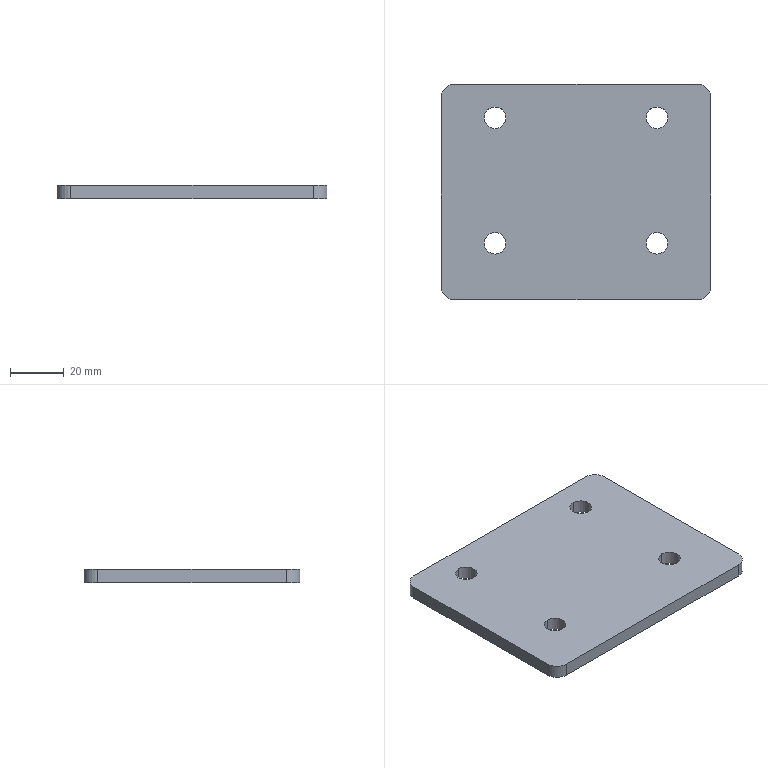Component | SolidWorks | VerticalMovingRectangularTubeWeldment-1_RectangularTubeWeldPlate1-2 | 1 solid | 18 faces | box 100 x 80 x 5 mm | volume 38887 mm3 | cylinder 12 | plane 6 | commonest cylinder face diameters 8 x8 10 x4 | material Plain Carbon Steel
STEP:
#1=CARTESIAN_POINT('',(11.024,-0.9055,-0.7874));
#2=VERTEX_POINT('',#1);
#3=CARTESIAN_POINT('',(11.024,-0.5906,-0.7874));
#4=VERTEX_POINT('',#3);
#5=CARTESIAN_POINT('',(11.024,-0.748,-0.7874));
#6=DIRECTION('',(0.,0.,-1.));
#7=DIRECTION('',(0.,1.,0.));
#8=AXIS2_PLACEMENT_3D('',#5,#6,#7);
#9=CIRCLE('',#8,0.1575);
#10=EDGE_CURVE('',#2,#4,#9,.T.);
#11=ORIENTED_EDGE('',*,*,#10,.F.);
#12=CARTESIAN_POINT('',(11.024,-0.9055,-0.9843));
#13=VERTEX_POINT('',#12);
#14=CARTESIAN_POINT('',(11.024,-0.9055,-0.9843));
#15=DIRECTION('',(0.,-0.,-1.));
#16=VECTOR('',#15,39.37);
#17=LINE('',#14,#16);
#18=EDGE_CURVE('',#2,#13,#17,.T.);
#19=ORIENTED_EDGE('',*,*,#18,.T.);
#20=CARTESIAN_POINT('',(11.024,-0.5906,-0.9843));
#21=VERTEX_POINT('',#20);
#22=CARTESIAN_POINT('',(11.024,-0.748,-0.9843));
#23=DIRECTION('',(0.,-0.,-1.));
#24=DIRECTION('',(0.,1.,0.));
#25=AXIS2_PLACEMENT_3D('',#22,#23,#24);
#26=CIRCLE('',#25,0.1575);
#27=EDGE_CURVE('',#13,#21,#26,.T.);
#28=ORIENTED_EDGE('',*,*,#27,.T.);
#29=CARTESIAN_POINT('',(11.024,-0.5906,-0.9843));
#30=DIRECTION('',(0.,-0.,-1.));
#31=VECTOR('',#30,39.37);
#32=LINE('',#29,#31);
#33=EDGE_CURVE('',#4,#21,#32,.T.);
#34=ORIENTED_EDGE('',*,*,#33,.F.);
#35=EDGE_LOOP('',(#11,#19,#28,#34));
#36=FACE_OUTER_BOUND('',#35,.T.);
#37=CARTESIAN_POINT('',(11.024,-0.748,-0.9843));
#38=DIRECTION('',(0.,-0.,-1.));
#39=DIRECTION('',(0.,1.,0.));
#40=AXIS2_PLACEMENT_3D('',#37,#38,#39);
#41=CYLINDRICAL_SURFACE('',#40,0.1575);
#42=ADVANCED_FACE('',(#36),#41,.F.);
#43=CARTESIAN_POINT('',(8.661,-0.9055,-0.7874));
#44=VERTEX_POINT('',#43);
#45=CARTESIAN_POINT('',(8.661,-0.5906,-0.7874));
#46=VERTEX_POINT('',#45);
#47=CARTESIAN_POINT('',(8.661,-0.748,-0.7874));
#48=DIRECTION('',(0.,0.,-1.));
#49=DIRECTION('',(0.,1.,0.));
#50=AXIS2_PLACEMENT_3D('',#47,#48,#49);
#51=CIRCLE('',#50,0.1575);
#52=EDGE_CURVE('',#44,#46,#51,.T.);
#53=ORIENTED_EDGE('',*,*,#52,.F.);
#54=CARTESIAN_POINT('',(8.661,-0.9055,-0.9843));
#55=VERTEX_POINT('',#54);
#56=CARTESIAN_POINT('',(8.661,-0.9055,-0.9843));
#57=DIRECTION('',(0.,-0.,-1.));
#58=VECTOR('',#57,39.37);
#59=LINE('',#56,#58);
#60=EDGE_CURVE('',#44,#55,#59,.T.);
#61=ORIENTED_EDGE('',*,*,#60,.T.);
#62=CARTESIAN_POINT('',(8.661,-0.5906,-0.9843));
#63=VERTEX_POINT('',#62);
#64=CARTESIAN_POINT('',(8.661,-0.748,-0.9843));
#65=DIRECTION('',(0.,-0.,-1.));
#66=DIRECTION('',(0.,1.,0.));
#67=AXIS2_PLACEMENT_3D('',#64,#65,#66);
#68=CIRCLE('',#67,0.1575);
#69=EDGE_CURVE('',#55,#63,#68,.T.);
#70=ORIENTED_EDGE('',*,*,#69,.T.);
#71=CARTESIAN_POINT('',(8.661,-0.5906,-0.9843));
#72=DIRECTION('',(0.,-0.,-1.));
#73=VECTOR('',#72,39.37);
#74=LINE('',#71,#73);
#75=EDGE_CURVE('',#46,#63,#74,.T.);
#76=ORIENTED_EDGE('',*,*,#75,.F.);
#77=EDGE_LOOP('',(#53,#61,#70,#76));
#78=FACE_OUTER_BOUND('',#77,.T.);
#79=CARTESIAN_POINT('',(8.661,-0.748,-0.9843));
#80=DIRECTION('',(0.,-0.,-1.));
#81=DIRECTION('',(0.,1.,0.));
#82=AXIS2_PLACEMENT_3D('',#79,#80,#81);
#83=CYLINDRICAL_SURFACE('',#82,0.1575);
#84=ADVANCED_FACE('',(#78),#83,.F.);
#85=CARTESIAN_POINT('',(11.024,0.9252,-0.7874));
#86=VERTEX_POINT('',#85);
#87=CARTESIAN_POINT('',(11.024,1.24,-0.7874));
#88=VERTEX_POINT('',#87);
#89=CARTESIAN_POINT('',(11.024,1.083,-0.7874));
#90=DIRECTION('',(0.,0.,-1.));
#91=DIRECTION('',(0.,1.,0.));
#92=AXIS2_PLACEMENT_3D('',#89,#90,#91);
#93=CIRCLE('',#92,0.1575);
#94=EDGE_CURVE('',#86,#88,#93,.T.);
#95=ORIENTED_EDGE('',*,*,#94,.F.);
#96=CARTESIAN_POINT('',(11.024,0.9252,-0.9843));
#97=VERTEX_POINT('',#96);
#98=CARTESIAN_POINT('',(11.024,0.9252,-0.9843));
#99=DIRECTION('',(0.,-0.,-1.));
#100=VECTOR('',#99,39.37);
#101=LINE('',#98,#100);
#102=EDGE_CURVE('',#86,#97,#101,.T.);
#103=ORIENTED_EDGE('',*,*,#102,.T.);
#104=CARTESIAN_POINT('',(11.024,1.24,-0.9843));
#105=VERTEX_POINT('',#104);
#106=CARTESIAN_POINT('',(11.024,1.083,-0.9843));
#107=DIRECTION('',(0.,-0.,-1.));
#108=DIRECTION('',(0.,1.,0.));
#109=AXIS2_PLACEMENT_3D('',#106,#107,#108);
#110=CIRCLE('',#109,0.1575);
#111=EDGE_CURVE('',#97,#105,#110,.T.);
#112=ORIENTED_EDGE('',*,*,#111,.T.);
#113=CARTESIAN_POINT('',(11.024,1.24,-0.9843));
#114=DIRECTION('',(0.,-0.,-1.));
#115=VECTOR('',#114,39.37);
#116=LINE('',#113,#115);
#117=EDGE_CURVE('',#88,#105,#116,.T.);
#118=ORIENTED_EDGE('',*,*,#117,.F.);
#119=EDGE_LOOP('',(#95,#103,#112,#118));
#120=FACE_OUTER_BOUND('',#119,.T.);
#121=CARTESIAN_POINT('',(11.024,1.083,-0.9843));
#122=DIRECTION('',(0.,-0.,-1.));
#123=DIRECTION('',(0.,1.,0.));
#124=AXIS2_PLACEMENT_3D('',#121,#122,#123);
#125=CYLINDRICAL_SURFACE('',#124,0.1575);
#126=ADVANCED_FACE('',(#120),#125,.F.);
#127=CARTESIAN_POINT('',(8.661,0.9252,-0.7874));
#128=VERTEX_POINT('',#127);
#129=CARTESIAN_POINT('',(8.661,1.24,-0.7874));
#130=VERTEX_POINT('',#129);
#131=CARTESIAN_POINT('',(8.661,1.083,-0.7874));
#132=DIRECTION('',(0.,0.,-1.));
#133=DIRECTION('',(0.,1.,0.));
#134=AXIS2_PLACEMENT_3D('',#131,#132,#133);
#135=CIRCLE('',#134,0.1575);
#136=EDGE_CURVE('',#128,#130,#135,.T.);
#137=ORIENTED_EDGE('',*,*,#136,.F.);
#138=CARTESIAN_POINT('',(8.661,0.9252,-0.9843));
#139=VERTEX_POINT('',#138);
#140=CARTESIAN_POINT('',(8.661,0.9252,-0.9843));
#141=DIRECTION('',(0.,-0.,-1.));
#142=VECTOR('',#141,39.37);
#143=LINE('',#140,#142);
#144=EDGE_CURVE('',#128,#139,#143,.T.);
#145=ORIENTED_EDGE('',*,*,#144,.T.);
#146=CARTESIAN_POINT('',(8.661,1.24,-0.9843));
#147=VERTEX_POINT('',#146);
#148=CARTESIAN_POINT('',(8.661,1.083,-0.9843));
#149=DIRECTION('',(0.,-0.,-1.));
#150=DIRECTION('',(0.,1.,0.));
#151=AXIS2_PLACEMENT_3D('',#148,#149,#150);
#152=CIRCLE('',#151,0.1575);
#153=EDGE_CURVE('',#139,#147,#152,.T.);
#154=ORIENTED_EDGE('',*,*,#153,.T.);
#155=CARTESIAN_POINT('',(8.661,1.24,-0.9843));
#156=DIRECTION('',(0.,-0.,-1.));
#157=VECTOR('',#156,39.37);
#158=LINE('',#155,#157);
#159=EDGE_CURVE('',#130,#147,#158,.T.);
#160=ORIENTED_EDGE('',*,*,#159,.F.);
#161=EDGE_LOOP('',(#137,#145,#154,#160));
#162=FACE_OUTER_BOUND('',#161,.T.);
#163=CARTESIAN_POINT('',(8.661,1.083,-0.9843));
#164=DIRECTION('',(0.,-0.,-1.));
#165=DIRECTION('',(0.,1.,0.));
#166=AXIS2_PLACEMENT_3D('',#163,#164,#165);
#167=CYLINDRICAL_SURFACE('',#166,0.1575);
#168=ADVANCED_FACE('',(#162),#167,.F.);
#169=CARTESIAN_POINT('',(11.811,-1.378,-0.7874));
#170=VERTEX_POINT('',#169);
#171=CARTESIAN_POINT('',(11.811,-1.378,-0.9843));
#172=VERTEX_POINT('',#171);
#173=CARTESIAN_POINT('',(11.811,-1.378,-0.7874));
#174=DIRECTION('',(0.,0.,-1.));
#175=VECTOR('',#174,39.37);
#176=LINE('',#173,#175);
#177=EDGE_CURVE('',#170,#172,#176,.T.);
#178=ORIENTED_EDGE('',*,*,#177,.T.);
#179=CARTESIAN_POINT('',(11.811,1.378,-0.9843));
#180=VERTEX_POINT('',#179);
#181=CARTESIAN_POINT('',(11.811,-1.575,-0.9843));
#182=DIRECTION('',(0.,1.,-0.));
#183=VECTOR('',#182,39.37);
#184=LINE('',#181,#183);
#185=EDGE_CURVE('',#172,#180,#184,.T.);
#186=ORIENTED_EDGE('',*,*,#185,.T.);
#187=CARTESIAN_POINT('',(11.811,1.378,-0.7874));
#188=VERTEX_POINT('',#187);
#189=CARTESIAN_POINT('',(11.811,1.378,-0.7874));
#190=DIRECTION('',(0.,0.,1.));
#191=VECTOR('',#190,39.37);
#192=LINE('',#189,#191);
#193=EDGE_CURVE('',#180,#188,#192,.T.);
#194=ORIENTED_EDGE('',*,*,#193,.T.);
#195=CARTESIAN_POINT('',(11.811,-1.575,-0.7874));
#196=DIRECTION('',(0.,1.,0.));
#197=VECTOR('',#196,39.37);
#198=LINE('',#195,#197);
#199=EDGE_CURVE('',#170,#188,#198,.T.);
#200=ORIENTED_EDGE('',*,*,#199,.F.);
#201=EDGE_LOOP('',(#178,#186,#194,#200));
#202=FACE_OUTER_BOUND('',#201,.T.);
#203=CARTESIAN_POINT('',(11.811,-1.575,-0.7874));
#204=DIRECTION('',(-1.,0.,0.));
#205=DIRECTION('',(0.,-1.,0.));
#206=AXIS2_PLACEMENT_3D('',#203,#204,#205);
#207=PLANE('',#206);
#208=ADVANCED_FACE('',(#202),#207,.F.);
#209=CARTESIAN_POINT('',(11.614,1.575,-0.7874));
#210=VERTEX_POINT('',#209);
#211=CARTESIAN_POINT('',(11.614,1.575,-0.9843));
#212=VERTEX_POINT('',#211);
#213=CARTESIAN_POINT('',(11.614,1.575,-0.7874));
#214=DIRECTION('',(0.,0.,-1.));
#215=VECTOR('',#214,39.37);
#216=LINE('',#213,#215);
#217=EDGE_CURVE('',#210,#212,#216,.T.);
#218=ORIENTED_EDGE('',*,*,#217,.T.);
#219=CARTESIAN_POINT('',(8.071,1.575,-0.9843));
#220=VERTEX_POINT('',#219);
#221=CARTESIAN_POINT('',(7.874,1.575,-0.9843));
#222=DIRECTION('',(-1.,0.,0.));
#223=VECTOR('',#222,39.37);
#224=LINE('',#221,#223);
#225=EDGE_CURVE('',#212,#220,#224,.T.);
#226=ORIENTED_EDGE('',*,*,#225,.T.);
#227=CARTESIAN_POINT('',(8.071,1.575,-0.7874));
#228=VERTEX_POINT('',#227);
#229=CARTESIAN_POINT('',(8.071,1.575,-0.7874));
#230=DIRECTION('',(0.,0.,1.));
#231=VECTOR('',#230,39.37);
#232=LINE('',#229,#231);
#233=EDGE_CURVE('',#220,#228,#232,.T.);
#234=ORIENTED_EDGE('',*,*,#233,.T.);
#235=CARTESIAN_POINT('',(7.874,1.575,-0.7874));
#236=DIRECTION('',(-1.,0.,0.));
#237=VECTOR('',#236,39.37);
#238=LINE('',#235,#237);
#239=EDGE_CURVE('',#210,#228,#238,.T.);
#240=ORIENTED_EDGE('',*,*,#239,.F.);
#241=EDGE_LOOP('',(#218,#226,#234,#240));
#242=FACE_OUTER_BOUND('',#241,.T.);
#243=CARTESIAN_POINT('',(7.874,1.575,-0.7874));
#244=DIRECTION('',(0.,-1.,0.));
#245=DIRECTION('',(1.,0.,0.));
#246=AXIS2_PLACEMENT_3D('',#243,#244,#245);
#247=PLANE('',#246);
#248=ADVANCED_FACE('',(#242),#247,.F.);
#249=CARTESIAN_POINT('',(7.874,1.378,-0.7874));
#250=VERTEX_POINT('',#249);
#251=CARTESIAN_POINT('',(7.874,1.378,-0.9843));
#252=VERTEX_POINT('',#251);
#253=CARTESIAN_POINT('',(7.874,1.378,-0.7874));
#254=DIRECTION('',(0.,0.,-1.));
#255=VECTOR('',#254,39.37);
#256=LINE('',#253,#255);
#257=EDGE_CURVE('',#250,#252,#256,.T.);
#258=ORIENTED_EDGE('',*,*,#257,.T.);
#259=CARTESIAN_POINT('',(7.874,-1.378,-0.9843));
#260=VERTEX_POINT('',#259);
#261=CARTESIAN_POINT('',(7.874,-1.575,-0.9843));
#262=DIRECTION('',(0.,-1.,0.));
#263=VECTOR('',#262,39.37);
#264=LINE('',#261,#263);
#265=EDGE_CURVE('',#252,#260,#264,.T.);
#266=ORIENTED_EDGE('',*,*,#265,.T.);
#267=CARTESIAN_POINT('',(7.874,-1.378,-0.7874));
#268=VERTEX_POINT('',#267);
#269=CARTESIAN_POINT('',(7.874,-1.378,-0.7874));
#270=DIRECTION('',(0.,0.,1.));
#271=VECTOR('',#270,39.37);
#272=LINE('',#269,#271);
#273=EDGE_CURVE('',#260,#268,#272,.T.);
#274=ORIENTED_EDGE('',*,*,#273,.T.);
#275=CARTESIAN_POINT('',(7.874,-1.575,-0.7874));
#276=DIRECTION('',(0.,-1.,0.));
#277=VECTOR('',#276,39.37);
#278=LINE('',#275,#277);
#279=EDGE_CURVE('',#250,#268,#278,.T.);
#280=ORIENTED_EDGE('',*,*,#279,.F.);
#281=EDGE_LOOP('',(#258,#266,#274,#280));
#282=FACE_OUTER_BOUND('',#281,.T.);
#283=CARTESIAN_POINT('',(7.874,-1.575,-0.7874));
#284=DIRECTION('',(1.,0.,0.));
#285=DIRECTION('',(0.,1.,0.));
#286=AXIS2_PLACEMENT_3D('',#283,#284,#285);
#287=PLANE('',#286);
#288=ADVANCED_FACE('',(#282),#287,.F.);
#289=CARTESIAN_POINT('',(8.071,-1.575,-0.7874));
#290=VERTEX_POINT('',#289);
#291=CARTESIAN_POINT('',(8.071,-1.575,-0.9843));
#292=VERTEX_POINT('',#291);
#293=CARTESIAN_POINT('',(8.071,-1.575,-0.7874));
#294=DIRECTION('',(0.,0.,-1.));
#295=VECTOR('',#294,39.37);
#296=LINE('',#293,#295);
#297=EDGE_CURVE('',#290,#292,#296,.T.);
#298=ORIENTED_EDGE('',*,*,#297,.T.);
#299=CARTESIAN_POINT('',(11.614,-1.575,-0.9843));
#300=VERTEX_POINT('',#299);
#301=CARTESIAN_POINT('',(7.874,-1.575,-0.9843));
#302=DIRECTION('',(1.,0.,0.));
#303=VECTOR('',#302,39.37);
#304=LINE('',#301,#303);
#305=EDGE_CURVE('',#292,#300,#304,.T.);
#306=ORIENTED_EDGE('',*,*,#305,.T.);
#307=CARTESIAN_POINT('',(11.614,-1.575,-0.7874));
#308=VERTEX_POINT('',#307);
#309=CARTESIAN_POINT('',(11.614,-1.575,-0.7874));
#310=DIRECTION('',(0.,0.,1.));
#311=VECTOR('',#310,39.37);
#312=LINE('',#309,#311);
#313=EDGE_CURVE('',#300,#308,#312,.T.);
#314=ORIENTED_EDGE('',*,*,#313,.T.);
#315=CARTESIAN_POINT('',(7.874,-1.575,-0.7874));
#316=DIRECTION('',(1.,0.,0.));
#317=VECTOR('',#316,39.37);
#318=LINE('',#315,#317);
#319=EDGE_CURVE('',#290,#308,#318,.T.);
#320=ORIENTED_EDGE('',*,*,#319,.F.);
#321=EDGE_LOOP('',(#298,#306,#314,#320));
#322=FACE_OUTER_BOUND('',#321,.T.);
#323=CARTESIAN_POINT('',(7.874,-1.575,-0.7874));
#324=DIRECTION('',(0.,1.,0.));
#325=DIRECTION('',(-1.,0.,0.));
#326=AXIS2_PLACEMENT_3D('',#323,#324,#325);
#327=PLANE('',#326);
#328=ADVANCED_FACE('',(#322),#327,.F.);
#329=CARTESIAN_POINT('',(11.024,-0.748,-0.7874));
#330=DIRECTION('',(0.,0.,-1.));
#331=DIRECTION('',(0.,1.,0.));
#332=AXIS2_PLACEMENT_3D('',#329,#330,#331);
#333=CIRCLE('',#332,0.1575);
#334=EDGE_CURVE('',#4,#2,#333,.T.);
#335=ORIENTED_EDGE('',*,*,#334,.T.);
#336=ORIENTED_EDGE('',*,*,#10,.T.);
#337=EDGE_LOOP('',(#335,#336));
#338=FACE_BOUND('',#337,.T.);
#339=CARTESIAN_POINT('',(8.661,-0.748,-0.7874));
#340=DIRECTION('',(0.,0.,-1.));
#341=DIRECTION('',(0.,1.,0.));
#342=AXIS2_PLACEMENT_3D('',#339,#340,#341);
#343=CIRCLE('',#342,0.1575);
#344=EDGE_CURVE('',#46,#44,#343,.T.);
#345=ORIENTED_EDGE('',*,*,#344,.T.);
#346=ORIENTED_EDGE('',*,*,#52,.T.);
#347=EDGE_LOOP('',(#345,#346));
#348=FACE_BOUND('',#347,.T.);
#349=CARTESIAN_POINT('',(11.024,1.083,-0.7874));
#350=DIRECTION('',(0.,0.,-1.));
#351=DIRECTION('',(0.,1.,0.));
#352=AXIS2_PLACEMENT_3D('',#349,#350,#351);
#353=CIRCLE('',#352,0.1575);
#354=EDGE_CURVE('',#88,#86,#353,.T.);
#355=ORIENTED_EDGE('',*,*,#354,.T.);
#356=ORIENTED_EDGE('',*,*,#94,.T.);
#357=EDGE_LOOP('',(#355,#356));
#358=FACE_BOUND('',#357,.T.);
#359=CARTESIAN_POINT('',(8.661,1.083,-0.7874));
#360=DIRECTION('',(0.,0.,-1.));
#361=DIRECTION('',(0.,1.,0.));
#362=AXIS2_PLACEMENT_3D('',#359,#360,#361);
#363=CIRCLE('',#362,0.1575);
#364=EDGE_CURVE('',#130,#128,#363,.T.);
#365=ORIENTED_EDGE('',*,*,#364,.T.);
#366=ORIENTED_EDGE('',*,*,#136,.T.);
#367=EDGE_LOOP('',(#365,#366));
#368=FACE_BOUND('',#367,.T.);
#369=ORIENTED_EDGE('',*,*,#199,.T.);
#370=CARTESIAN_POINT('',(11.614,1.378,-0.7874));
#371=DIRECTION('',(0.,0.,1.));
#372=DIRECTION('',(0.,1.,0.));
#373=AXIS2_PLACEMENT_3D('',#370,#371,#372);
#374=CIRCLE('',#373,0.1969);
#375=EDGE_CURVE('',#188,#210,#374,.T.);
#376=ORIENTED_EDGE('',*,*,#375,.T.);
#377=ORIENTED_EDGE('',*,*,#239,.T.);
#378=CARTESIAN_POINT('',(8.071,1.378,-0.7874));
#379=DIRECTION('',(0.,0.,1.));
#380=DIRECTION('',(0.,1.,0.));
#381=AXIS2_PLACEMENT_3D('',#378,#379,#380);
#382=CIRCLE('',#381,0.1969);
#383=EDGE_CURVE('',#228,#250,#382,.T.);
#384=ORIENTED_EDGE('',*,*,#383,.T.);
#385=ORIENTED_EDGE('',*,*,#279,.T.);
#386=CARTESIAN_POINT('',(8.071,-1.378,-0.7874));
#387=DIRECTION('',(0.,0.,1.));
#388=DIRECTION('',(0.,1.,0.));
#389=AXIS2_PLACEMENT_3D('',#386,#387,#388);
#390=CIRCLE('',#389,0.1969);
#391=EDGE_CURVE('',#268,#290,#390,.T.);
#392=ORIENTED_EDGE('',*,*,#391,.T.);
#393=ORIENTED_EDGE('',*,*,#319,.T.);
#394=CARTESIAN_POINT('',(11.614,-1.378,-0.7874));
#395=DIRECTION('',(0.,0.,1.));
#396=DIRECTION('',(0.,1.,0.));
#397=AXIS2_PLACEMENT_3D('',#394,#395,#396);
#398=CIRCLE('',#397,0.1969);
#399=EDGE_CURVE('',#308,#170,#398,.T.);
#400=ORIENTED_EDGE('',*,*,#399,.T.);
#401=EDGE_LOOP('',(#369,#376,#377,#384,#385,#392,#393,#400));
#402=FACE_OUTER_BOUND('',#401,.T.);
#403=CARTESIAN_POINT('',(9.843,0.,-0.7874));
#404=DIRECTION('',(0.,0.,-1.));
#405=DIRECTION('',(0.,1.,0.));
#406=AXIS2_PLACEMENT_3D('',#403,#404,#405);
#407=PLANE('',#406);
#408=ADVANCED_FACE('',(#338,#348,#358,#368,#402),#407,.F.);
#409=CARTESIAN_POINT('',(11.614,1.378,-0.9843));
#410=DIRECTION('',(0.,-0.,-1.));
#411=DIRECTION('',(0.,-1.,0.));
#412=AXIS2_PLACEMENT_3D('',#409,#410,#411);
#413=CIRCLE('',#412,0.1969);
#414=EDGE_CURVE('',#212,#180,#413,.T.);
#415=ORIENTED_EDGE('',*,*,#414,.F.);
#416=ORIENTED_EDGE('',*,*,#217,.F.);
#417=ORIENTED_EDGE('',*,*,#375,.F.);
#418=ORIENTED_EDGE('',*,*,#193,.F.);
#419=EDGE_LOOP('',(#415,#416,#417,#418));
#420=FACE_OUTER_BOUND('',#419,.T.);
#421=CARTESIAN_POINT('',(11.614,1.378,-0.7874));
#422=DIRECTION('',(0.,0.,-1.));
#423=DIRECTION('',(0.,1.,0.));
#424=AXIS2_PLACEMENT_3D('',#421,#422,#423);
#425=CYLINDRICAL_SURFACE('',#424,0.1969);
#426=ADVANCED_FACE('',(#420),#425,.T.);
#427=CARTESIAN_POINT('',(11.614,-1.378,-0.9843));
#428=DIRECTION('',(0.,-0.,-1.));
#429=DIRECTION('',(0.,-1.,0.));
#430=AXIS2_PLACEMENT_3D('',#427,#428,#429);
#431=CIRCLE('',#430,0.1969);
#432=EDGE_CURVE('',#172,#300,#431,.T.);
#433=ORIENTED_EDGE('',*,*,#432,.F.);
#434=ORIENTED_EDGE('',*,*,#177,.F.);
#435=ORIENTED_EDGE('',*,*,#399,.F.);
#436=ORIENTED_EDGE('',*,*,#313,.F.);
#437=EDGE_LOOP('',(#433,#434,#435,#436));
#438=FACE_OUTER_BOUND('',#437,.T.);
#439=CARTESIAN_POINT('',(11.614,-1.378,-0.7874));
#440=DIRECTION('',(0.,0.,-1.));
#441=DIRECTION('',(0.,1.,0.));
#442=AXIS2_PLACEMENT_3D('',#439,#440,#441);
#443=CYLINDRICAL_SURFACE('',#442,0.1969);
#444=ADVANCED_FACE('',(#438),#443,.T.);
#445=CARTESIAN_POINT('',(8.071,-1.378,-0.9843));
#446=DIRECTION('',(0.,-0.,-1.));
#447=DIRECTION('',(0.,-1.,0.));
#448=AXIS2_PLACEMENT_3D('',#445,#446,#447);
#449=CIRCLE('',#448,0.1969);
#450=EDGE_CURVE('',#292,#260,#449,.T.);
#451=ORIENTED_EDGE('',*,*,#450,.F.);
#452=ORIENTED_EDGE('',*,*,#297,.F.);
#453=ORIENTED_EDGE('',*,*,#391,.F.);
#454=ORIENTED_EDGE('',*,*,#273,.F.);
#455=EDGE_LOOP('',(#451,#452,#453,#454));
#456=FACE_OUTER_BOUND('',#455,.T.);
#457=CARTESIAN_POINT('',(8.071,-1.378,-0.7874));
#458=DIRECTION('',(0.,0.,-1.));
#459=DIRECTION('',(0.,1.,0.));
#460=AXIS2_PLACEMENT_3D('',#457,#458,#459);
#461=CYLINDRICAL_SURFACE('',#460,0.1969);
#462=ADVANCED_FACE('',(#456),#461,.T.);
#463=CARTESIAN_POINT('',(8.071,1.378,-0.9843));
#464=DIRECTION('',(0.,-0.,-1.));
#465=DIRECTION('',(0.,-1.,0.));
#466=AXIS2_PLACEMENT_3D('',#463,#464,#465);
#467=CIRCLE('',#466,0.1969);
#468=EDGE_CURVE('',#252,#220,#467,.T.);
#469=ORIENTED_EDGE('',*,*,#468,.F.);
#470=ORIENTED_EDGE('',*,*,#257,.F.);
#471=ORIENTED_EDGE('',*,*,#383,.F.);
#472=ORIENTED_EDGE('',*,*,#233,.F.);
#473=EDGE_LOOP('',(#469,#470,#471,#472));
#474=FACE_OUTER_BOUND('',#473,.T.);
#475=CARTESIAN_POINT('',(8.071,1.378,-0.7874));
#476=DIRECTION('',(0.,0.,-1.));
#477=DIRECTION('',(0.,1.,0.));
#478=AXIS2_PLACEMENT_3D('',#475,#476,#477);
#479=CYLINDRICAL_SURFACE('',#478,0.1969);
#480=ADVANCED_FACE('',(#474),#479,.T.);
#481=CARTESIAN_POINT('',(11.024,-0.748,-0.9843));
#482=DIRECTION('',(0.,-0.,-1.));
#483=DIRECTION('',(0.,1.,0.));
#484=AXIS2_PLACEMENT_3D('',#481,#482,#483);
#485=CIRCLE('',#484,0.1575);
#486=EDGE_CURVE('',#21,#13,#485,.T.);
#487=ORIENTED_EDGE('',*,*,#486,.F.);
#488=ORIENTED_EDGE('',*,*,#27,.F.);
#489=EDGE_LOOP('',(#487,#488));
#490=FACE_BOUND('',#489,.T.);
#491=CARTESIAN_POINT('',(8.661,-0.748,-0.9843));
#492=DIRECTION('',(0.,-0.,-1.));
#493=DIRECTION('',(0.,1.,0.));
#494=AXIS2_PLACEMENT_3D('',#491,#492,#493);
#495=CIRCLE('',#494,0.1575);
#496=EDGE_CURVE('',#63,#55,#495,.T.);
#497=ORIENTED_EDGE('',*,*,#496,.F.);
#498=ORIENTED_EDGE('',*,*,#69,.F.);
#499=EDGE_LOOP('',(#497,#498));
#500=FACE_BOUND('',#499,.T.);
#501=CARTESIAN_POINT('',(11.024,1.083,-0.9843));
#502=DIRECTION('',(0.,-0.,-1.));
#503=DIRECTION('',(0.,1.,0.));
#504=AXIS2_PLACEMENT_3D('',#501,#502,#503);
#505=CIRCLE('',#504,0.1575);
#506=EDGE_CURVE('',#105,#97,#505,.T.);
#507=ORIENTED_EDGE('',*,*,#506,.F.);
#508=ORIENTED_EDGE('',*,*,#111,.F.);
#509=EDGE_LOOP('',(#507,#508));
#510=FACE_BOUND('',#509,.T.);
#511=CARTESIAN_POINT('',(8.661,1.083,-0.9843));
#512=DIRECTION('',(0.,-0.,-1.));
#513=DIRECTION('',(0.,1.,0.));
#514=AXIS2_PLACEMENT_3D('',#511,#512,#513);
#515=CIRCLE('',#514,0.1575);
#516=EDGE_CURVE('',#147,#139,#515,.T.);
#517=ORIENTED_EDGE('',*,*,#516,.F.);
#518=ORIENTED_EDGE('',*,*,#153,.F.);
#519=EDGE_LOOP('',(#517,#518));
#520=FACE_BOUND('',#519,.T.);
#521=ORIENTED_EDGE('',*,*,#432,.T.);
#522=ORIENTED_EDGE('',*,*,#305,.F.);
#523=ORIENTED_EDGE('',*,*,#450,.T.);
#524=ORIENTED_EDGE('',*,*,#265,.F.);
#525=ORIENTED_EDGE('',*,*,#468,.T.);
#526=ORIENTED_EDGE('',*,*,#225,.F.);
#527=ORIENTED_EDGE('',*,*,#414,.T.);
#528=ORIENTED_EDGE('',*,*,#185,.F.);
#529=EDGE_LOOP('',(#521,#522,#523,#524,#525,#526,#527,#528));
#530=FACE_OUTER_BOUND('',#529,.T.);
#531=CARTESIAN_POINT('',(20.079,2.218,-0.9843));
#532=DIRECTION('',(0.,0.,1.));
#533=DIRECTION('',(0.,-1.,0.));
#534=AXIS2_PLACEMENT_3D('',#531,#532,#533);
#535=PLANE('',#534);
#536=ADVANCED_FACE('',(#490,#500,#510,#520,#530),#535,.F.);
#537=ORIENTED_EDGE('',*,*,#144,.F.);
#538=ORIENTED_EDGE('',*,*,#364,.F.);
#539=ORIENTED_EDGE('',*,*,#159,.T.);
#540=ORIENTED_EDGE('',*,*,#516,.T.);
#541=EDGE_LOOP('',(#537,#538,#539,#540));
#542=FACE_OUTER_BOUND('',#541,.T.);
#543=CARTESIAN_POINT('',(8.661,1.083,-0.9843));
#544=DIRECTION('',(0.,-0.,-1.));
#545=DIRECTION('',(0.,1.,0.));
#546=AXIS2_PLACEMENT_3D('',#543,#544,#545);
#547=CYLINDRICAL_SURFACE('',#546,0.1575);
#548=ADVANCED_FACE('',(#542),#547,.F.);
#549=ORIENTED_EDGE('',*,*,#102,.F.);
#550=ORIENTED_EDGE('',*,*,#354,.F.);
#551=ORIENTED_EDGE('',*,*,#117,.T.);
#552=ORIENTED_EDGE('',*,*,#506,.T.);
#553=EDGE_LOOP('',(#549,#550,#551,#552));
#554=FACE_OUTER_BOUND('',#553,.T.);
#555=CARTESIAN_POINT('',(11.024,1.083,-0.9843));
#556=DIRECTION('',(0.,-0.,-1.));
#557=DIRECTION('',(0.,1.,0.));
#558=AXIS2_PLACEMENT_3D('',#555,#556,#557);
#559=CYLINDRICAL_SURFACE('',#558,0.1575);
#560=ADVANCED_FACE('',(#554),#559,.F.);
#561=ORIENTED_EDGE('',*,*,#60,.F.);
#562=ORIENTED_EDGE('',*,*,#344,.F.);
#563=ORIENTED_EDGE('',*,*,#75,.T.);
#564=ORIENTED_EDGE('',*,*,#496,.T.);
#565=EDGE_LOOP('',(#561,#562,#563,#564));
#566=FACE_OUTER_BOUND('',#565,.T.);
#567=CARTESIAN_POINT('',(8.661,-0.748,-0.9843));
#568=DIRECTION('',(0.,-0.,-1.));
#569=DIRECTION('',(0.,1.,0.));
#570=AXIS2_PLACEMENT_3D('',#567,#568,#569);
#571=CYLINDRICAL_SURFACE('',#570,0.1575);
#572=ADVANCED_FACE('',(#566),#571,.F.);
#573=ORIENTED_EDGE('',*,*,#18,.F.);
#574=ORIENTED_EDGE('',*,*,#334,.F.);
#575=ORIENTED_EDGE('',*,*,#33,.T.);
#576=ORIENTED_EDGE('',*,*,#486,.T.);
#577=EDGE_LOOP('',(#573,#574,#575,#576));
#578=FACE_OUTER_BOUND('',#577,.T.);
#579=CARTESIAN_POINT('',(11.024,-0.748,-0.9843));
#580=DIRECTION('',(0.,-0.,-1.));
#581=DIRECTION('',(0.,1.,0.));
#582=AXIS2_PLACEMENT_3D('',#579,#580,#581);
#583=CYLINDRICAL_SURFACE('',#582,0.1575);
#584=ADVANCED_FACE('',(#578),#583,.F.);
#585=CLOSED_SHELL('',(#42,#84,#126,#168,#208,#248,#288,#328,#408,#426,#444,#462,#480,#536,#548,#560,#572,#584));
#586=MANIFOLD_SOLID_BREP('',#585);
#587=CARTESIAN_POINT('',(0.,0.,0.));
#588=DIRECTION('',(0.,0.,1.));
#589=DIRECTION('',(1.,0.,0.));
#590=AXIS2_PLACEMENT_3D('',#587,#588,#589);
#591=(LENGTH_UNIT()NAMED_UNIT(*)SI_UNIT($,.METRE.));
#592=LENGTH_MEASURE_WITH_UNIT(LENGTH_MEASURE(0.0254),#591);
#593=DIMENSIONAL_EXPONENTS(1.,0.,0.,0.,0.,0.,0.);
#594=(CONVERSION_BASED_UNIT('',#592)LENGTH_UNIT()NAMED_UNIT(#593));
#595=UNCERTAINTY_MEASURE_WITH_UNIT(LENGTH_MEASURE(0.00001),#594,'','');
#596=(NAMED_UNIT(*)PLANE_ANGLE_UNIT()SI_UNIT($,.RADIAN.));
#597=(NAMED_UNIT(*)SI_UNIT($,.STERADIAN.)SOLID_ANGLE_UNIT());
#598=(GEOMETRIC_REPRESENTATION_CONTEXT(3)GLOBAL_UNCERTAINTY_ASSIGNED_CONTEXT((#595))GLOBAL_UNIT_ASSIGNED_CONTEXT((#594,#596,#597))REPRESENTATION_CONTEXT('',''));
#599=ADVANCED_BREP_SHAPE_REPRESENTATION('',(#586,#590),#598);
#600=COLOUR_RGB('',0.7922,0.8196,0.9333);
#601=FILL_AREA_STYLE_COLOUR('',#600);
#602=FILL_AREA_STYLE('',(#601));
#603=SURFACE_STYLE_FILL_AREA(#602);
#604=SURFACE_SIDE_STYLE('',(#603));
#605=SURFACE_STYLE_USAGE(.BOTH.,#604);
#606=PRESENTATION_STYLE_ASSIGNMENT((#605));
#607=STYLED_ITEM('',(#606),#586);
#608=(LENGTH_UNIT()NAMED_UNIT(*)SI_UNIT($,.METRE.));
#609=LENGTH_MEASURE_WITH_UNIT(LENGTH_MEASURE(0.0254),#608);
#610=DIMENSIONAL_EXPONENTS(1.,0.,0.,0.,0.,0.,0.);
#611=(CONVERSION_BASED_UNIT('',#609)LENGTH_UNIT()NAMED_UNIT(#610));
#612=UNCERTAINTY_MEASURE_WITH_UNIT(LENGTH_MEASURE(0.00001),#611,'','');
#613=(NAMED_UNIT(*)PLANE_ANGLE_UNIT()SI_UNIT($,.RADIAN.));
#614=(NAMED_UNIT(*)SI_UNIT($,.STERADIAN.)SOLID_ANGLE_UNIT());
#615=(GEOMETRIC_REPRESENTATION_CONTEXT(3)GLOBAL_UNCERTAINTY_ASSIGNED_CONTEXT((#612))GLOBAL_UNIT_ASSIGNED_CONTEXT((#611,#613,#614))REPRESENTATION_CONTEXT('',''));
#616=MECHANICAL_DESIGN_GEOMETRIC_PRESENTATION_REPRESENTATION('',(#607),#615);
#617=PRESENTATION_LAYER_ASSIGNMENT('','',(#607));